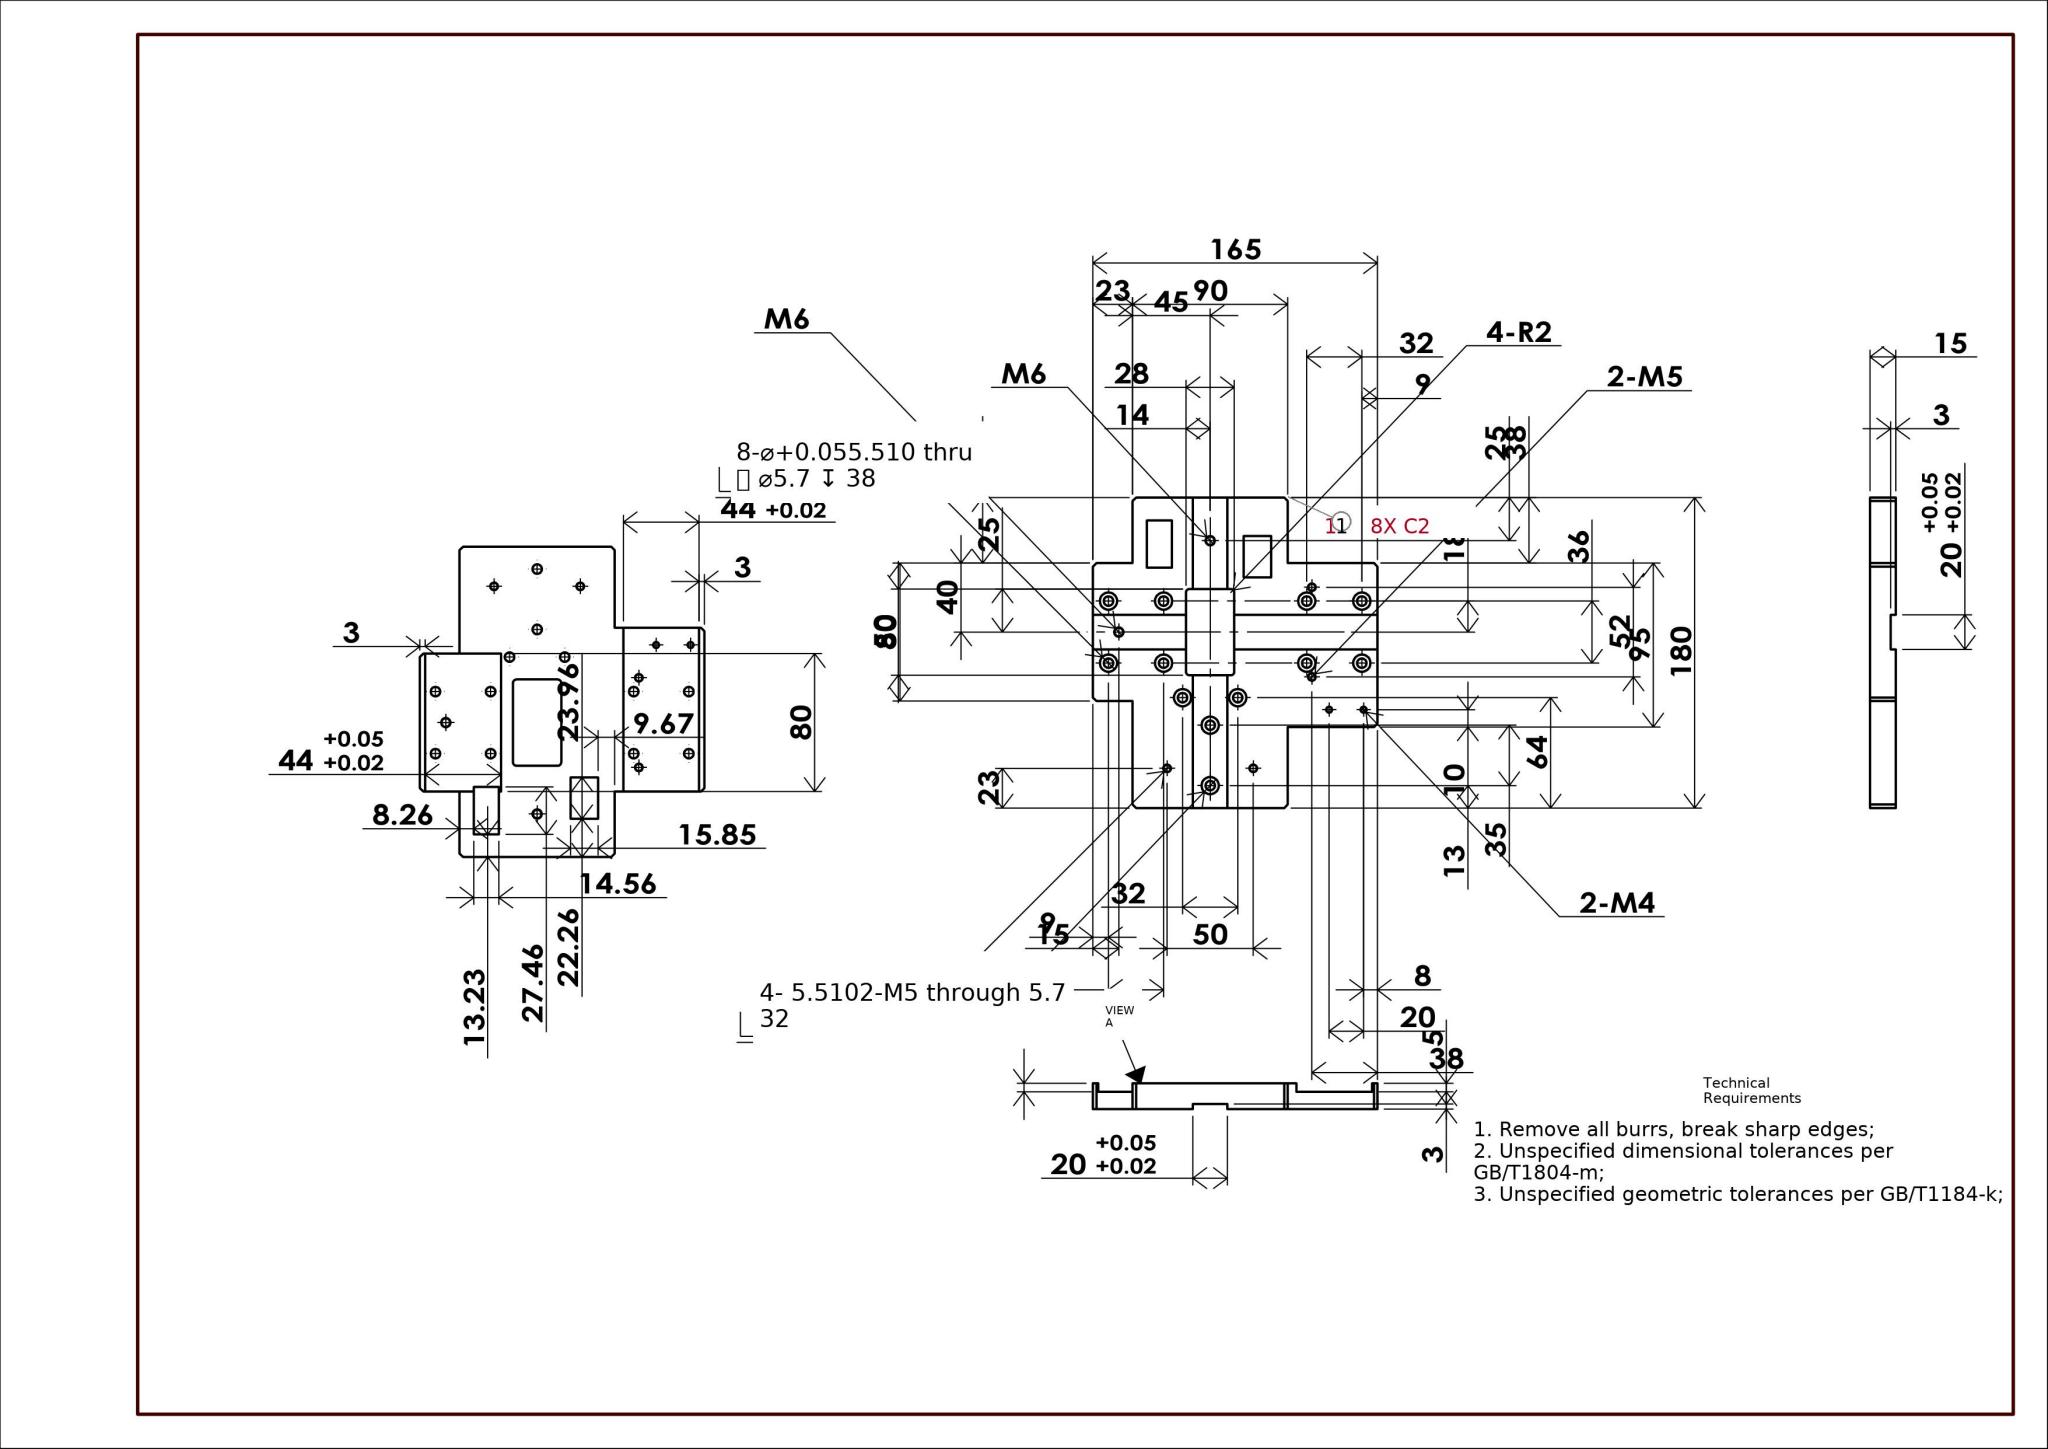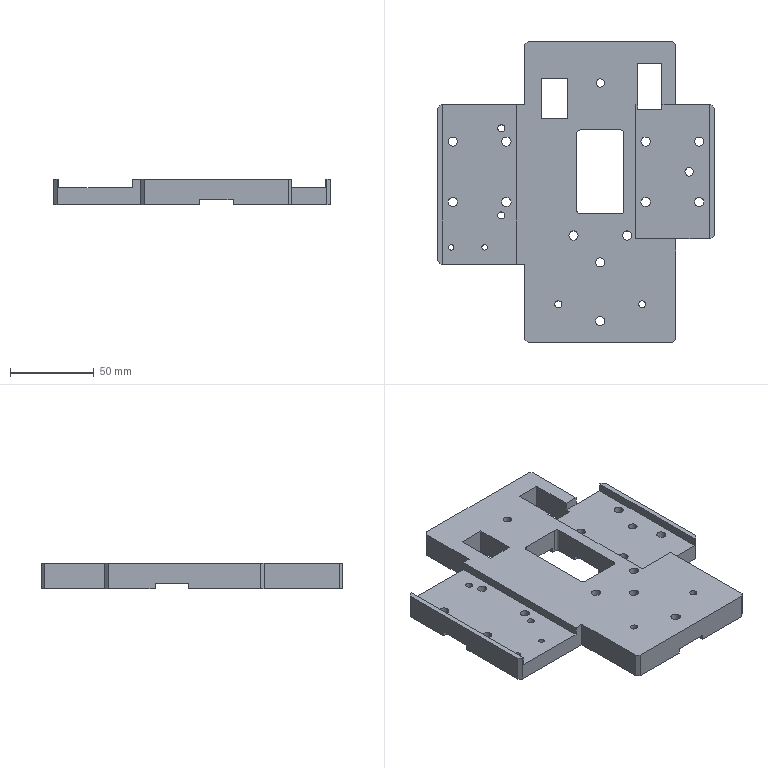Part | SolidWorks | mm | 1 solid | 140 faces | box 165 x 180 x 15 mm | volume 249324 mm3 | plane 72 | cylinder 68 | commonest cylinder face diameters 10 x24 5.5 x24 4.2 x8 3.3 x4 5 x4 4 x4